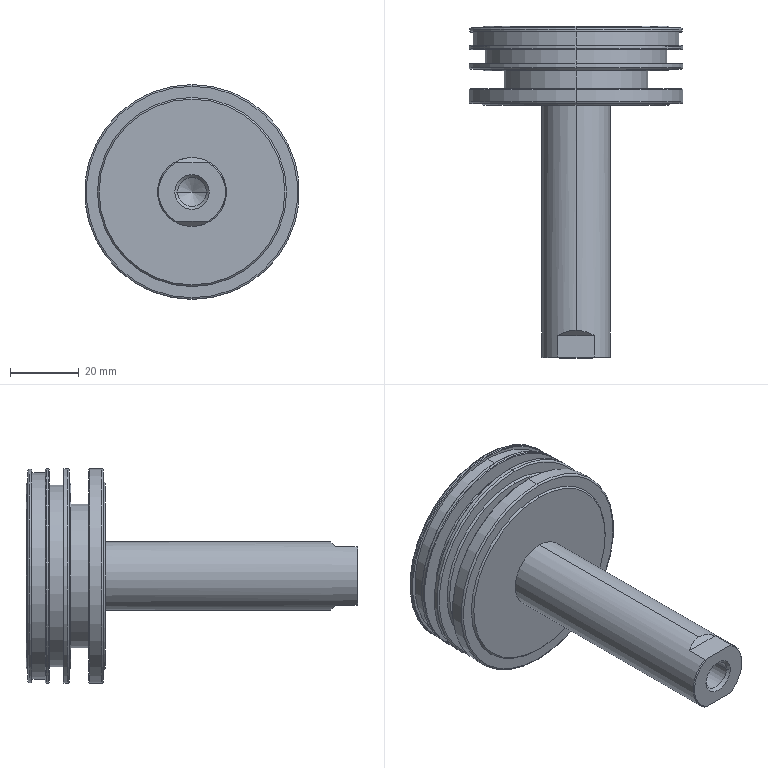Component | SolidWorks | ACQS_63x50_G_2_50-1_ACQS_63x50_50r-1 | 1 solid | 62 faces | box 62.5 x 96.5 x 62.5 mm | volume 78014 mm3 | cone 22 | cylinder 18 | plane 16 | torus 6 | commonest cylinder face diameters 62.5 x6 8.376 x2 62.1 x2 60 x2 52.9 x2 41.8 x2 20 x2
build123d program:
from build123d import *

# Parameters (mm, degrees)
CUT_EXTRUDE1_DEPTH      = 17
CUT_EXTRUDE1_DEPTH_BACK = 17


with BuildPart() as part:
    # Sketch1 → Revolve1 (revolve)
    with BuildSketch(Plane.XY, mode=Mode.PRIVATE) as revolve1_sk:
        Polygon((-8, 0), (-8, 9.75), (-7.75, 10), (0, 10), (0, 0), align=None)
    revolve(revolve1_sk.sketch.rotate(Axis((0, 0, 0), (-1, 0, 0)), 270), axis=Axis((0, 0, 0), (-1, 0, 0)))

    # Sketch2 → Revolve2 (revolve)
    with BuildSketch(Plane.XY, mode=Mode.PRIVATE) as revolve2_sk:
        with BuildLine():
            Line((0, 0), (0, 10))
            Line((0, 10), (65.5, 10))
            Line((65.5, 10), (65.5, 27))
            Line((65.5, 27), (66, 27.5))
            Line((66, 27.5), (66, 30.75))
            ThreePointArc((66, 30.75), (66.146, 31.104), (66.5, 31.25))
            Line((66.5, 31.25), (70, 31.25))
            Line((70, 31.25), (70.3, 30.95))
            Line((70.3, 30.95), (70.3, 20.9))
            Line((70.3, 20.9), (75.5, 20.9))
            Line((75.5, 20.9), (75.5, 27))
            Line((75.5, 27), (76, 27.5))
            Line((76, 27.5), (76, 30.75))
            ThreePointArc((76, 30.75), (76.146, 31.104), (76.5, 31.25))
            Line((76.5, 31.25), (77.5, 31.25))
            Line((77.5, 31.25), (77.7, 31.05))
            Line((77.7, 31.05), (77.7, 26.45))
            Line((77.7, 26.45), (81.7, 26.45))
            Line((81.7, 26.45), (81.7, 31.05))
            Line((81.7, 31.05), (81.9, 31.25))
            Line((81.9, 31.25), (82.7, 31.25))
            Line((82.7, 31.25), (82.9, 31.05))
            Line((82.9, 31.05), (82.9, 30))
            Line((82.9, 30), (86.8, 30))
            Line((86.8, 30), (86.8, 30.85))
            Line((86.8, 30.85), (87, 31.05))
            Line((87, 31.05), (87.5, 31.05))
            ThreePointArc((87.5, 31.05), (87.854, 30.904), (88, 30.55))
            Line((88, 30.55), (88, 27.5))
            Line((88, 27.5), (88.5, 27))
            Line((88.5, 27), (88.5, 0))
            Line((88.5, 0), (0, 0))
        make_face()
    revolve(revolve2_sk.sketch.rotate(Axis((88.5, 0, 0), (-1, 0, 0)), 270), axis=Axis((88.5, 0, 0), (-1, 0, 0)))

    # Sketch3 → Cut-Extrude1 (cut, two sides: drawn at the far end of the back side and taken through both)
    with BuildSketch(Plane(origin=(0, 0, 0), x_dir=(1, 0, 0), z_dir=(0, 1, 0)).offset(-CUT_EXTRUDE1_DEPTH_BACK)):
        Polygon((-18, -13.5), (3.5, -13.5), (-1.5, -8.5), (-8, -8.5), (-8, 8.5), (-1.5, 8.5), (3.5, 13.5), (-18, 13.5), align=None)
    extrude(amount=CUT_EXTRUDE1_DEPTH + CUT_EXTRUDE1_DEPTH_BACK, mode=Mode.SUBTRACT)

    # Sketch4 → Cut-Revolve1 (revolve, cut)
    with BuildSketch(Plane.XY, mode=Mode.PRIVATE) as cut_revolve1_sk:
        Polygon((-8, 0), (-8, 5), (-7.188, 4.188), (10, 4.188), (12.418, 0), align=None)
    revolve(cut_revolve1_sk.sketch.rotate(Axis((12.418, 0, 0), (-1, 0, 0)), 180), axis=Axis((12.418, 0, 0), (-1, 0, 0)), mode=Mode.SUBTRACT)


solid = part.part

# Placed as in the assembly
solid = solid.moved(Location((-566.612, -300.873, 2398.4), (0, 0, 90)))